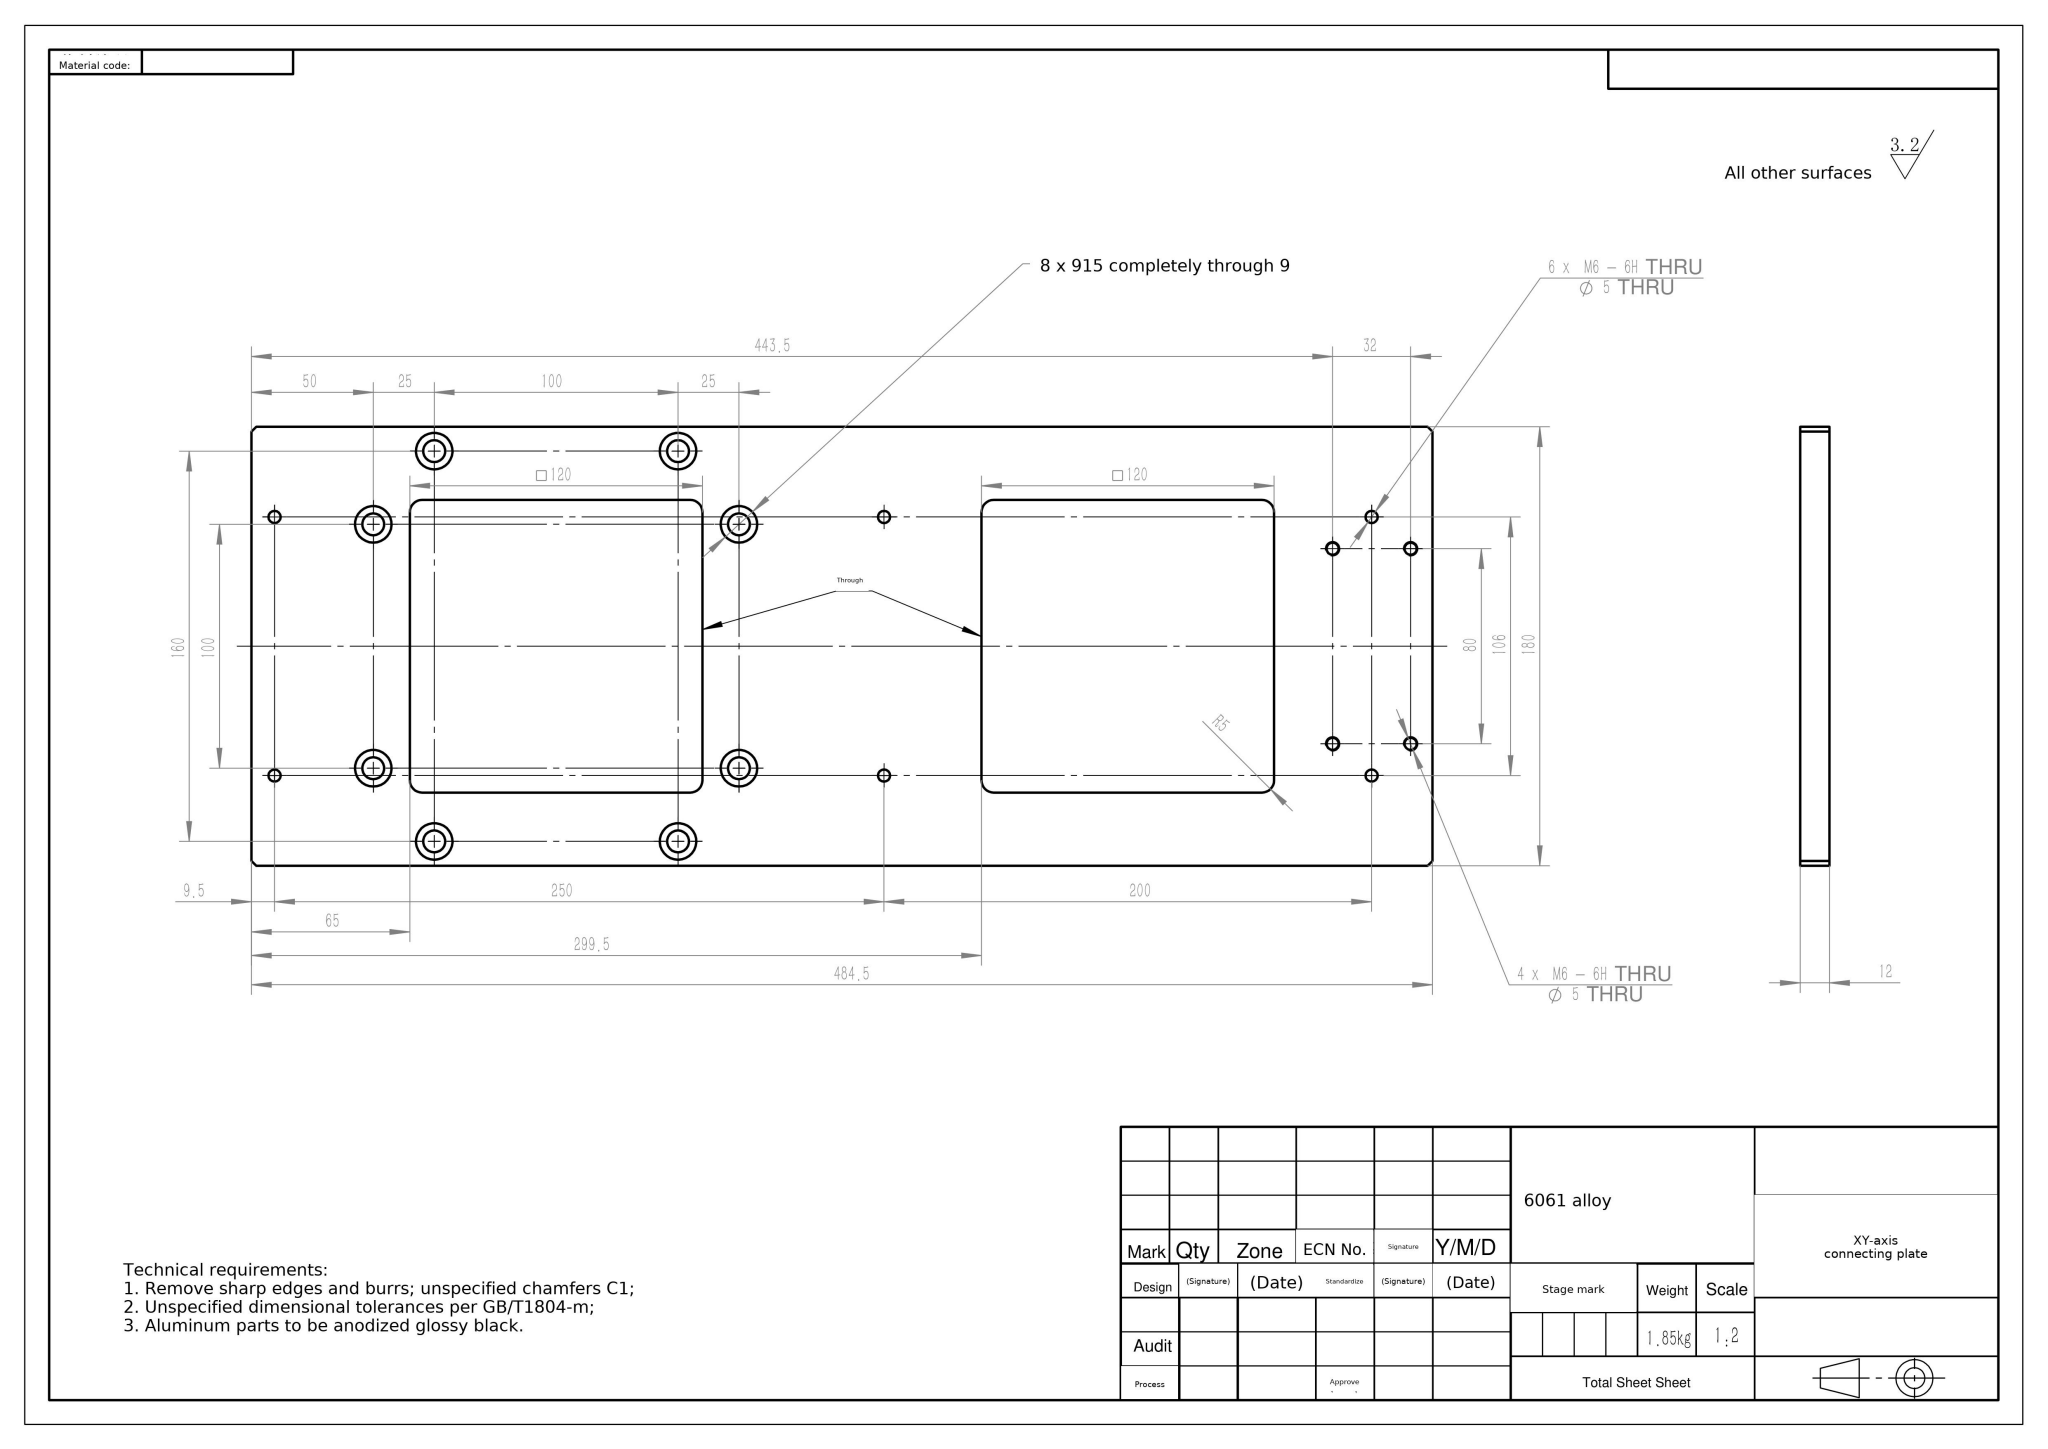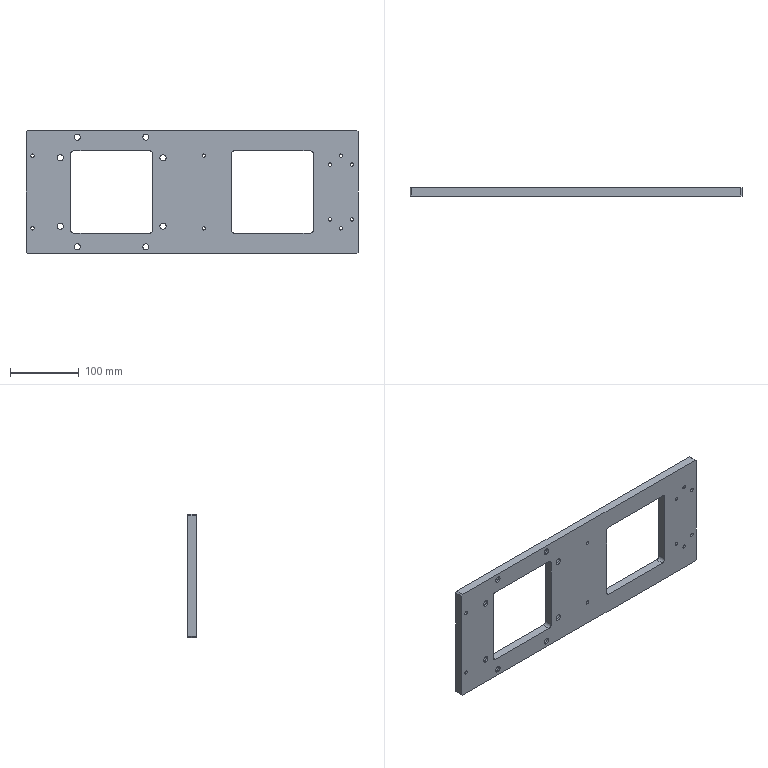Part | SolidWorks | mm | material 6061 alloy | 1 solid | 86 faces | box 484.5 x 12 x 180 mm | volume 684733 mm3 | cylinder 60 | plane 26 | commonest cylinder face diameters 5 x20 15 x16 9 x16 10 x8
build123d program:
from build123d import *

# Parameters (mm, degrees)
SKETCH1_W                                          = 484.5
SKETCH1_H                                          = 180
BOSS_EXTRUDE1_DEPTH                                = 12
HOLE_SIZE_ACCORDING_TO_TYPE_0_OF_HEX_S_D           = 9
HOLE_SIZE_ACCORDING_TO_TYPE_0_OF_HEX_S_CBORE_D     = 15
HOLE_SIZE_ACCORDING_TO_TYPE_0_OF_HEX_S_CBORE_DEPTH = 9
M6_TAPPED_HOLE1_D                                  = 5
M6_TAPPED_HOLE2_D                                  = 5
CHAMFER1_SIZE                                      = 2
CUT_EXTRUDE1_DEPTH                                 = 259.707


with BuildPart() as part:
    # Sketch1 → Boss-Extrude1 (new body)
    with BuildSketch(Plane(origin=(0, 0, 0), x_dir=(1, 0, 0), z_dir=(0, 1, 0))):
        Rectangle(SKETCH1_W, SKETCH1_H)
    extrude(amount=BOSS_EXTRUDE1_DEPTH)

    # Hole Size _according to_ Type 0 of Hex S (through all)
    with Locations(Plane(origin=(0, 12, 0), x_dir=(1, 0, 0), z_dir=(0, 1, 0))):
        with Locations((-167.25, 80), (-67.25, 80), (-192.25, 50), (-42.25, 50), (-42.25, -50), (-192.25, -50), (-67.25, -80), (-167.25, -80)):
            CounterBoreHole(HOLE_SIZE_ACCORDING_TO_TYPE_0_OF_HEX_S_D / 2, HOLE_SIZE_ACCORDING_TO_TYPE_0_OF_HEX_S_CBORE_D / 2, HOLE_SIZE_ACCORDING_TO_TYPE_0_OF_HEX_S_CBORE_DEPTH)

    # M6 Tapped Hole1 (through all)
    with Locations(Plane(origin=(0, 12, 0), x_dir=(1, 0, 0), z_dir=(0, 1, 0))):
        with Locations((-232.75, 53), (17.25, 53), (217.25, 53), (217.25, -53), (17.25, -53), (-232.75, -53)):
            Hole(M6_TAPPED_HOLE1_D / 2)

    # M6 Tapped Hole2 (through all)
    with Locations(Plane(origin=(0, 0, 0), x_dir=(-1, 0, 0), z_dir=(0, -1, 0))):
        with Locations((-201.25, -40), (-233.25, -40), (-201.25, 40), (-233.25, 40)):
            Hole(M6_TAPPED_HOLE2_D / 2)

    # Chamfer1
    chamfer1_edges = [part.edges().sort_by_distance(p)[0] for p in [
        (242.25, 6, 90),
        (-242.25, 6, 90),
        (-242.25, 6, -90),
        (242.25, 6, -90),
    ]]
    chamfer(chamfer1_edges, length=CHAMFER1_SIZE)

    # Sketch8 → Cut-Extrude1 (cut, through all)
    with BuildSketch(Plane.XZ):
        with BuildLine():
            Line((62.25, 60), (172.25, 60))
            ThreePointArc((172.25, 60), (175.786, 58.536), (177.25, 55))
            Line((177.25, 55), (177.25, -55))
            ThreePointArc((177.25, -55), (175.786, -58.536), (172.25, -60))
            Line((172.25, -60), (62.25, -60))
            ThreePointArc((62.25, -60), (58.714, -58.536), (57.25, -55))
            Line((57.25, -55), (57.25, 55))
            ThreePointArc((57.25, 55), (58.714, 58.536), (62.25, 60))
        make_face()
        with BuildLine():
            Line((-177.25, 55), (-177.25, -55))
            ThreePointArc((-177.25, -55), (-175.786, -58.536), (-172.25, -60))
            Line((-172.25, -60), (-62.25, -60))
            ThreePointArc((-62.25, -60), (-58.714, -58.536), (-57.25, -55))
            Line((-57.25, -55), (-57.25, 55))
            ThreePointArc((-57.25, 55), (-58.714, 58.536), (-62.25, 60))
            Line((-62.25, 60), (-172.25, 60))
            ThreePointArc((-172.25, 60), (-175.786, 58.536), (-177.25, 55))
        make_face()
    extrude(amount=-CUT_EXTRUDE1_DEPTH, mode=Mode.SUBTRACT)


solid = part.part